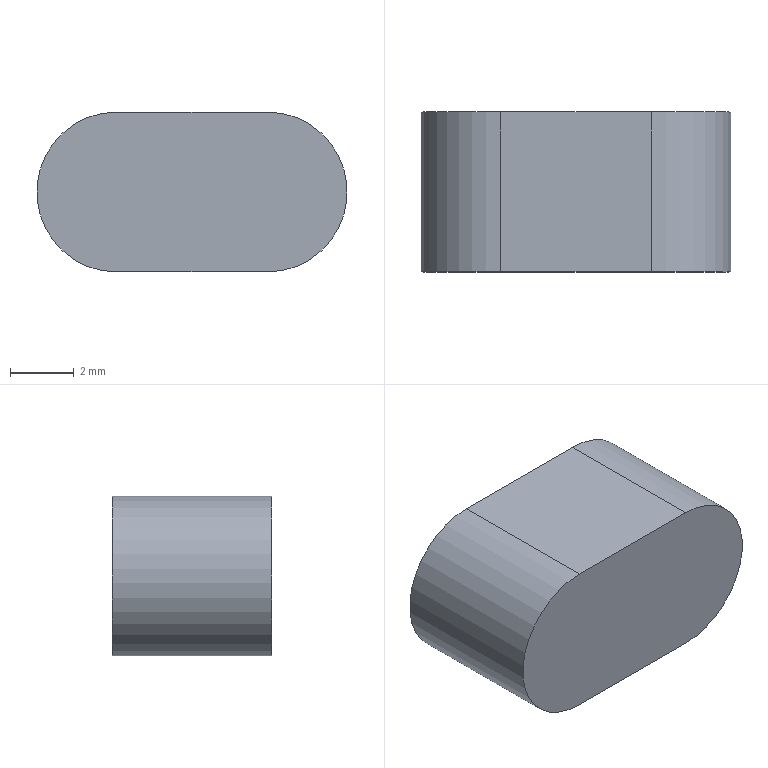Component | NX | KEY | 1 solid | 6 faces | volume 216 mm3 | plane 4 | cylinder 2 | commonest cylinder face diameters 5 x2